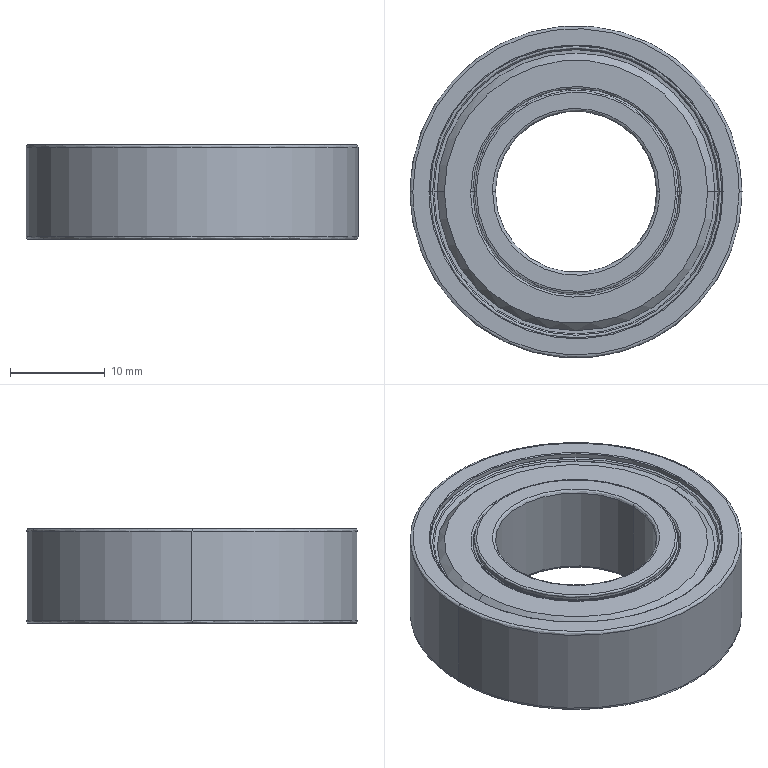Component | SolidWorks | BAU6003Z-2 | 1 solid | 82 faces | volume 5936 mm3 | spline 32 | cylinder 22 | cone 20 | plane 8 | commonest cylinder face diameters 29.4 x4 22.6 x4 35 x2 30.8 x2 17 x2 21.4 x2 20.6 x2 21.8 x2